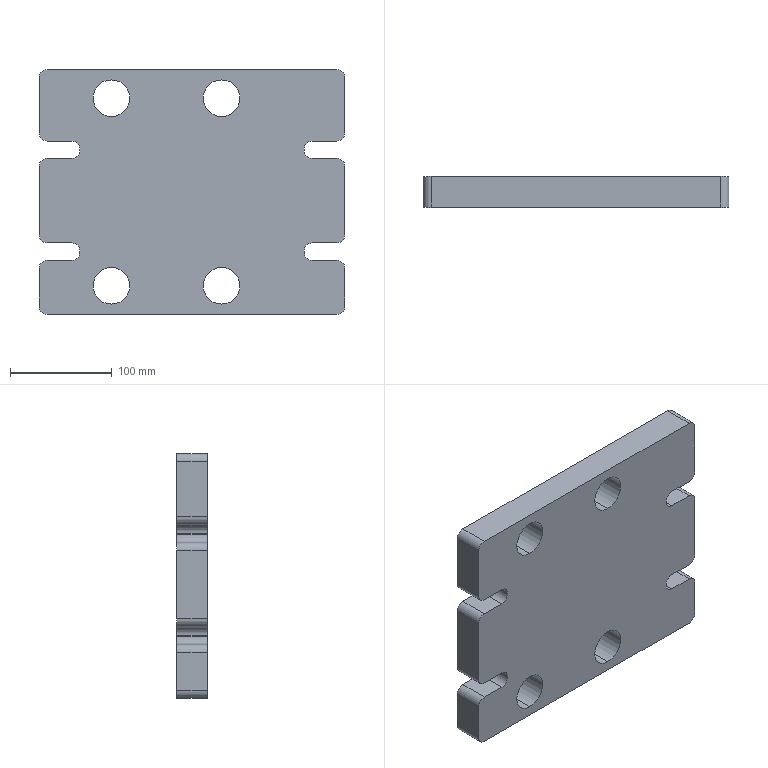Component | SolidWorks | Box151Fixture-1 | 1 solid | 158 faces | box 300 x 30 x 240 mm | volume 1941668 mm3 | cylinder 84 | cone 48 | plane 26 | commonest cylinder face diameters 3.3 x32 16 x20 6.8 x16 8 x8 36 x8
build123d program:
from build123d import *

# Parameters (mm, degrees)
SKETCH1_W             = 300
SKETCH1_H             = 240
BOSS_EXTRUDE1_DEPTH   = 30
SKETCH2_R             = 18
CUT_EXTRUDE1_DEPTH    = 50
M4_TAPPED_HOLE1_D     = 3.3
M4_TAPPED_HOLE1_DEPTH = 25
M4_TAPPED_HOLE1_TIP   = 0.9914
SKETCH5_R             = 4
CUT_EXTRUDE2_DEPTH    = 10
M8_TAPPED_HOLE1_D     = 6.8
M8_TAPPED_HOLE1_DEPTH = 25
M8_TAPPED_HOLE1_TIP   = 2.043
MOVE_FACE1_BY         = 40
MOVE_FACE2_BY         = 40
SKETCH9_W             = 40
SKETCH9_H             = 17
CUT_EXTRUDE3_DEPTH    = 30
FILLET1_R             = 8


with BuildPart() as part:
    # Sketch1 → Boss-Extrude1 (new body)
    with BuildSketch(Plane(origin=(0, 0, 0), x_dir=(1, 0, 0), z_dir=(0, 1, 0))):
        Rectangle(SKETCH1_W, SKETCH1_H)
    extrude(amount=BOSS_EXTRUDE1_DEPTH)

    # Sketch2 → Cut-Extrude1 (cut)
    with BuildSketch(Plane(origin=(0, 30, 0), x_dir=(1, 0, 0), z_dir=(0, 1, 0))):
        with Locations(Location((-119, -92, 0), (0, 0, 270))):
            Circle(SKETCH2_R)
        with Locations(Location((-11, -92, 0), (0, 0, 270))):
            Circle(SKETCH2_R)
        with Locations(Location((-11, 92, 0), (0, 0, 270))):
            Circle(SKETCH2_R)
        with Locations(Location((-119, 92, 0), (0, 0, 270))):
            Circle(SKETCH2_R)
    extrude(amount=-CUT_EXTRUDE1_DEPTH, mode=Mode.SUBTRACT)

    # M4 Tapped Hole1
    with Locations(Plane(origin=(0, 30, 0), x_dir=(1, 0, 0), z_dir=(0, 1, 0))):
        with Locations((-134.7, -76.3), (-103.3, -76.3), (-103.3, -107.7), (-134.7, -107.7), (-26.7, -76.3), (4.7, -76.3), (4.7, -107.7), (-26.7, -107.7), (-134.7, 107.7), (-134.7, 76.3), (-103.3, 107.7), (-103.3, 76.3), (-26.7, 107.7), (4.7, 107.7), (4.7, 76.3), (-26.7, 76.3)):
            Hole(M4_TAPPED_HOLE1_D / 2, depth=M4_TAPPED_HOLE1_DEPTH)
            with Locations((0, 0, -(M4_TAPPED_HOLE1_DEPTH + M4_TAPPED_HOLE1_TIP / 2))):  # 118° drill point
                Cone(0, M4_TAPPED_HOLE1_D / 2, M4_TAPPED_HOLE1_TIP, mode=Mode.SUBTRACT)

    # Sketch5 → Cut-Extrude2 (cut)
    with BuildSketch(Plane(origin=(0, 30, 0), x_dir=(1, 0, 0), z_dir=(0, 1, 0))):
        with Locations(Location((24.5, -62, 0), (0, 0, 270))):
            Circle(SKETCH5_R)
        with Locations(Location((-134.5, -38, 0), (0, 0, 270))):
            Circle(SKETCH5_R)
        with Locations(Location((-134.5, 62, 0), (0, 0, 270))):
            Circle(SKETCH5_R)
        with Locations(Location((24.5, 38, 0), (0, 0, 270))):
            Circle(SKETCH5_R)
    extrude(amount=-CUT_EXTRUDE2_DEPTH, mode=Mode.SUBTRACT)

    # M8 Tapped Hole1
    with Locations(Plane(origin=(0, 30, 0), x_dir=(1, 0, 0), z_dir=(0, 1, 0))):
        with Locations((-90, 50), (-55, 50), (-20, 50), (15, 50), (-20, -50), (-55, -50), (-90, -50), (-125, -50)):
            Hole(M8_TAPPED_HOLE1_D / 2, depth=M8_TAPPED_HOLE1_DEPTH)
            with Locations((0, 0, -(M8_TAPPED_HOLE1_DEPTH + M8_TAPPED_HOLE1_TIP / 2))):  # 118° drill point
                Cone(0, M8_TAPPED_HOLE1_D / 2, M8_TAPPED_HOLE1_TIP, mode=Mode.SUBTRACT)

    # Move Face1: a face moved inward by 40.0
    extrude(part.faces().sort_by_distance((150, 15, 0))[0], amount=MOVE_FACE1_BY, dir=(-1, 0, 0), mode=Mode.SUBTRACT)

    # Move Face2: a face moved outward by 40.0
    extrude(part.faces().sort_by_distance((-150, 15, 0))[0], amount=MOVE_FACE2_BY, dir=(-1, 0, 0))

    # Sketch9 → Cut-Extrude3 (cut)
    with BuildSketch(Plane(origin=(0, 30, 0), x_dir=(1, 0, 0), z_dir=(0, 1, 0))):
        with Locations((-170, 58.5)):
            Rectangle(SKETCH9_W, SKETCH9_H)
        with Locations((-170, -41.5)):
            Rectangle(SKETCH9_W, SKETCH9_H)
        with Locations((90, 58.5)):
            Rectangle(SKETCH9_W, SKETCH9_H)
        with Locations((90, -41.5)):
            Rectangle(SKETCH9_W, SKETCH9_H)
    extrude(amount=-CUT_EXTRUDE3_DEPTH, mode=Mode.SUBTRACT)

    # Fillet1
    fillet1_edges = [part.edges().sort_by_distance(p)[0] for p in [
        (-150, 15, 33),
        (-150, 15, 50),
        (-190, 15, 50),
        (-190, 15, 33),
        (110, 15, -67),
        (110, 15, -50),
        (70, 15, -50),
        (70, 15, -67),
        (110, 15, 33),
        (110, 15, 50),
        (70, 15, 50),
        (70, 15, 33),
        (-150, 15, -67),
        (-150, 15, -50),
        (-190, 15, -50),
        (-190, 15, -67),
        (110, 15, 120),
        (-190, 15, 120),
        (-190, 15, -120),
        (110, 15, -120),
    ]]
    fillet(fillet1_edges, radius=FILLET1_R)


solid = part.part

# Placed as in the assembly
solid = solid.moved(Location((51.381, 34.047, 0), (0, 0, 0)))